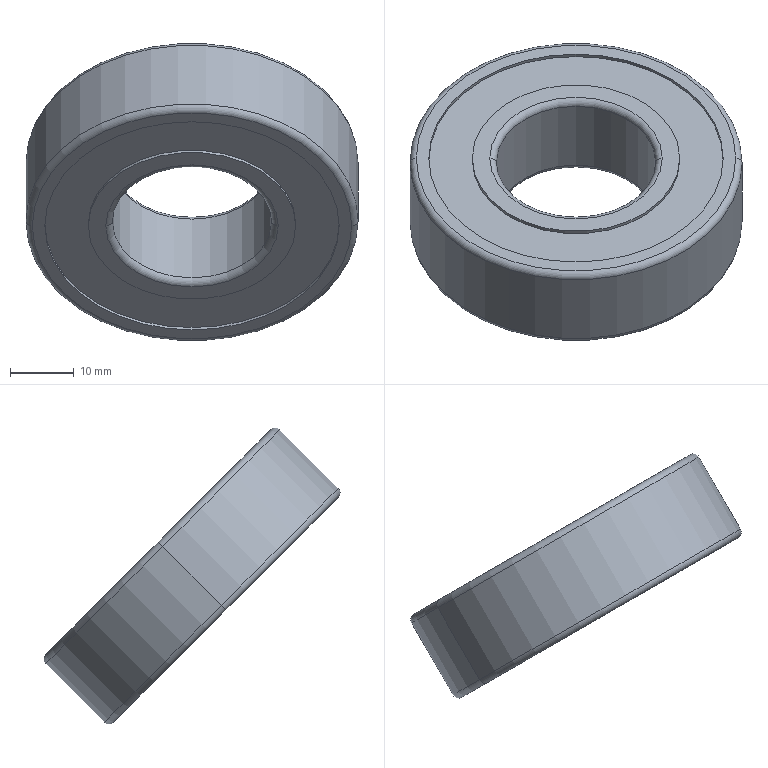Component | SolidWorks | PassiveRollerAssembly-1_Bearing6205-3 | 1 solid | 26 faces | box 52 x 46.55 x 46.55 mm | volume 23499 mm3 | cylinder 12 | torus 8 | plane 6 | commonest cylinder face diameters 46.1 x4 32.5 x4 52 x2 25 x2
build123d program:
from build123d import *


with BuildPart() as part:
    # Sketch1 → Revolve1 (revolve)
    with BuildSketch(Plane.XY, mode=Mode.PRIVATE) as revolve1_sk:
        with BuildLine():
            Line((0, 25), (0, 23.05))
            Line((0, 23.05), (0.53, 23.05))
            Line((0.53, 23.05), (0.53, 16.25))
            Line((0.53, 16.25), (0, 16.25))
            Line((0, 16.25), (0, 13.5))
            ThreePointArc((0, 13.5), (0.2929, 12.793), (1, 12.5))
            Line((1, 12.5), (14, 12.5))
            ThreePointArc((14, 12.5), (14.707, 12.793), (15, 13.5))
            Line((15, 13.5), (15, 16.25))
            Line((15, 16.25), (14.47, 16.25))
            Line((14.47, 16.25), (14.47, 23.05))
            Line((14.47, 23.05), (15, 23.05))
            Line((15, 23.05), (15, 25))
            ThreePointArc((15, 25), (14.707, 25.707), (14, 26))
            Line((14, 26), (1, 26))
            ThreePointArc((1, 26), (0.2929, 25.707), (0, 25))
        make_face()
    revolve(revolve1_sk.sketch.rotate(Axis((15, 0, 0), (-1, 0, 0)), 270), axis=Axis((15, 0, 0), (-1, 0, 0)))


solid = part.part

# Placed as in the assembly
solid = solid.moved(Location((2216.026, 747.574, 381.188), (-135, 89.432, 90)))
STEP:
#1=COLOUR_RGB('',0.7922,0.8196,0.9333);
#2=FILL_AREA_STYLE_COLOUR('',#1);
#3=FILL_AREA_STYLE('',(#2));
#4=SURFACE_STYLE_FILL_AREA(#3);
#5=SURFACE_SIDE_STYLE('',(#4));
#6=SURFACE_STYLE_USAGE(.BOTH.,#5);
#7=PRESENTATION_STYLE_ASSIGNMENT((#6));
#8=CARTESIAN_POINT('',(88.269,29.042,14.618));
#9=VERTEX_POINT('',#8);
#10=CARTESIAN_POINT('',(86.222,29.042,14.618));
#11=VERTEX_POINT('',#10);
#12=CARTESIAN_POINT('',(87.245,29.042,14.618));
#13=DIRECTION('',(-0.,0.7071,0.7071));
#14=DIRECTION('',(1.,0.,0.));
#15=AXIS2_PLACEMENT_3D('',#12,#13,#14);
#16=CIRCLE('',#15,1.024);
#17=EDGE_CURVE('',#9,#11,#16,.T.);
#18=ORIENTED_EDGE('',*,*,#17,.T.);
#19=CARTESIAN_POINT('',(86.222,29.404,14.98));
#20=VERTEX_POINT('',#19);
#21=CARTESIAN_POINT('',(86.222,29.014,14.59));
#22=DIRECTION('',(-0.,0.7071,0.7071));
#23=VECTOR('',#22,39.37);
#24=LINE('',#21,#23);
#25=EDGE_CURVE('',#11,#20,#24,.T.);
#26=ORIENTED_EDGE('',*,*,#25,.T.);
#27=CARTESIAN_POINT('',(88.269,29.404,14.98));
#28=VERTEX_POINT('',#27);
#29=CARTESIAN_POINT('',(87.245,29.404,14.98));
#30=DIRECTION('',(-0.,0.7071,0.7071));
#31=DIRECTION('',(1.,0.,0.));
#32=AXIS2_PLACEMENT_3D('',#29,#30,#31);
#33=CIRCLE('',#32,1.024);
#34=EDGE_CURVE('',#28,#20,#33,.T.);
#35=ORIENTED_EDGE('',*,*,#34,.F.);
#36=CARTESIAN_POINT('',(88.269,29.014,14.59));
#37=DIRECTION('',(-0.,0.7071,0.7071));
#38=VECTOR('',#37,39.37);
#39=LINE('',#36,#38);
#40=EDGE_CURVE('',#9,#28,#39,.T.);
#41=ORIENTED_EDGE('',*,*,#40,.F.);
#42=EDGE_LOOP('',(#18,#26,#35,#41));
#43=FACE_OUTER_BOUND('',#42,.T.);
#44=CARTESIAN_POINT('',(87.245,29.014,14.59));
#45=DIRECTION('',(-0.,0.7071,0.7071));
#46=DIRECTION('',(1.,0.,0.));
#47=AXIS2_PLACEMENT_3D('',#44,#45,#46);
#48=CYLINDRICAL_SURFACE('',#47,1.024);
#49=ADVANCED_FACE('',(#43),#48,.T.);
#50=CARTESIAN_POINT('',(88.229,29.014,14.59));
#51=VERTEX_POINT('',#50);
#52=CARTESIAN_POINT('',(86.261,29.014,14.59));
#53=VERTEX_POINT('',#52);
#54=CARTESIAN_POINT('',(87.245,29.014,14.59));
#55=DIRECTION('',(-0.,0.7071,0.7071));
#56=DIRECTION('',(1.,0.,0.));
#57=AXIS2_PLACEMENT_3D('',#54,#55,#56);
#58=CIRCLE('',#57,0.9843);
#59=EDGE_CURVE('',#51,#53,#58,.T.);
#60=ORIENTED_EDGE('',*,*,#59,.T.);
#61=CARTESIAN_POINT('',(86.261,29.042,14.618));
#62=DIRECTION('',(0.,0.7071,-0.7071));
#63=DIRECTION('',(0.,0.7071,0.7071));
#64=AXIS2_PLACEMENT_3D('',#61,#62,#63);
#65=CIRCLE('',#64,0.03937);
#66=EDGE_CURVE('',#53,#11,#65,.T.);
#67=ORIENTED_EDGE('',*,*,#66,.T.);
#68=ORIENTED_EDGE('',*,*,#17,.F.);
#69=CARTESIAN_POINT('',(88.229,29.042,14.618));
#70=DIRECTION('',(-0.,-0.7071,0.7071));
#71=DIRECTION('',(0.,-0.7071,-0.7071));
#72=AXIS2_PLACEMENT_3D('',#69,#70,#71);
#73=CIRCLE('',#72,0.03937);
#74=EDGE_CURVE('',#51,#9,#73,.T.);
#75=ORIENTED_EDGE('',*,*,#74,.F.);
#76=EDGE_LOOP('',(#60,#67,#68,#75));
#77=FACE_OUTER_BOUND('',#76,.T.);
#78=CARTESIAN_POINT('',(87.245,29.042,14.618));
#79=DIRECTION('',(-0.,0.7071,0.7071));
#80=DIRECTION('',(1.,0.,0.));
#81=AXIS2_PLACEMENT_3D('',#78,#79,#80);
#82=TOROIDAL_SURFACE('',#81,0.9843,0.03937);
#83=ADVANCED_FACE('',(#77),#82,.T.);
#84=CARTESIAN_POINT('',(86.338,29.014,14.59));
#85=VERTEX_POINT('',#84);
#86=CARTESIAN_POINT('',(88.153,29.014,14.59));
#87=VERTEX_POINT('',#86);
#88=CARTESIAN_POINT('',(87.245,29.014,14.59));
#89=DIRECTION('',(-0.,0.7071,0.7071));
#90=DIRECTION('',(1.,0.,0.));
#91=AXIS2_PLACEMENT_3D('',#88,#89,#90);
#92=CIRCLE('',#91,0.9075);
#93=EDGE_CURVE('',#85,#87,#92,.T.);
#94=ORIENTED_EDGE('',*,*,#93,.F.);
#95=CARTESIAN_POINT('',(86.338,29.029,14.605));
#96=VERTEX_POINT('',#95);
#97=CARTESIAN_POINT('',(86.338,29.014,14.59));
#98=DIRECTION('',(-0.,0.7071,0.7071));
#99=VECTOR('',#98,39.37);
#100=LINE('',#97,#99);
#101=EDGE_CURVE('',#85,#96,#100,.T.);
#102=ORIENTED_EDGE('',*,*,#101,.T.);
#103=CARTESIAN_POINT('',(88.153,29.029,14.605));
#104=VERTEX_POINT('',#103);
#105=CARTESIAN_POINT('',(87.245,29.029,14.605));
#106=DIRECTION('',(-0.,0.7071,0.7071));
#107=DIRECTION('',(1.,0.,0.));
#108=AXIS2_PLACEMENT_3D('',#105,#106,#107);
#109=CIRCLE('',#108,0.9075);
#110=EDGE_CURVE('',#96,#104,#109,.T.);
#111=ORIENTED_EDGE('',*,*,#110,.T.);
#112=CARTESIAN_POINT('',(88.153,29.014,14.59));
#113=DIRECTION('',(-0.,0.7071,0.7071));
#114=VECTOR('',#113,39.37);
#115=LINE('',#112,#114);
#116=EDGE_CURVE('',#87,#104,#115,.T.);
#117=ORIENTED_EDGE('',*,*,#116,.F.);
#118=EDGE_LOOP('',(#94,#102,#111,#117));
#119=FACE_OUTER_BOUND('',#118,.T.);
#120=CARTESIAN_POINT('',(87.245,29.014,14.59));
#121=DIRECTION('',(-0.,0.7071,0.7071));
#122=DIRECTION('',(1.,0.,0.));
#123=AXIS2_PLACEMENT_3D('',#120,#121,#122);
#124=CYLINDRICAL_SURFACE('',#123,0.9075);
#125=ADVANCED_FACE('',(#119),#124,.F.);
#126=CARTESIAN_POINT('',(87.885,29.014,14.59));
#127=VERTEX_POINT('',#126);
#128=CARTESIAN_POINT('',(86.605,29.014,14.59));
#129=VERTEX_POINT('',#128);
#130=CARTESIAN_POINT('',(87.245,29.014,14.59));
#131=DIRECTION('',(-0.,0.7071,0.7071));
#132=DIRECTION('',(1.,0.,0.));
#133=AXIS2_PLACEMENT_3D('',#130,#131,#132);
#134=CIRCLE('',#133,0.6398);
#135=EDGE_CURVE('',#127,#129,#134,.T.);
#136=ORIENTED_EDGE('',*,*,#135,.T.);
#137=CARTESIAN_POINT('',(86.605,29.029,14.605));
#138=VERTEX_POINT('',#137);
#139=CARTESIAN_POINT('',(86.605,29.014,14.59));
#140=DIRECTION('',(-0.,0.7071,0.7071));
#141=VECTOR('',#140,39.37);
#142=LINE('',#139,#141);
#143=EDGE_CURVE('',#129,#138,#142,.T.);
#144=ORIENTED_EDGE('',*,*,#143,.T.);
#145=CARTESIAN_POINT('',(87.885,29.029,14.605));
#146=VERTEX_POINT('',#145);
#147=CARTESIAN_POINT('',(87.245,29.029,14.605));
#148=DIRECTION('',(-0.,0.7071,0.7071));
#149=DIRECTION('',(1.,0.,0.));
#150=AXIS2_PLACEMENT_3D('',#147,#148,#149);
#151=CIRCLE('',#150,0.6398);
#152=EDGE_CURVE('',#146,#138,#151,.T.);
#153=ORIENTED_EDGE('',*,*,#152,.F.);
#154=CARTESIAN_POINT('',(87.885,29.014,14.59));
#155=DIRECTION('',(-0.,0.7071,0.7071));
#156=VECTOR('',#155,39.37);
#157=LINE('',#154,#156);
#158=EDGE_CURVE('',#127,#146,#157,.T.);
#159=ORIENTED_EDGE('',*,*,#158,.F.);
#160=EDGE_LOOP('',(#136,#144,#153,#159));
#161=FACE_OUTER_BOUND('',#160,.T.);
#162=CARTESIAN_POINT('',(87.245,29.014,14.59));
#163=DIRECTION('',(-0.,0.7071,0.7071));
#164=DIRECTION('',(1.,0.,0.));
#165=AXIS2_PLACEMENT_3D('',#162,#163,#164);
#166=CYLINDRICAL_SURFACE('',#165,0.6398);
#167=ADVANCED_FACE('',(#161),#166,.T.);
#168=CARTESIAN_POINT('',(87.737,29.042,14.618));
#169=VERTEX_POINT('',#168);
#170=CARTESIAN_POINT('',(86.753,29.042,14.618));
#171=VERTEX_POINT('',#170);
#172=CARTESIAN_POINT('',(87.245,29.042,14.618));
#173=DIRECTION('',(-0.,0.7071,0.7071));
#174=DIRECTION('',(1.,0.,0.));
#175=AXIS2_PLACEMENT_3D('',#172,#173,#174);
#176=CIRCLE('',#175,0.4921);
#177=EDGE_CURVE('',#169,#171,#176,.T.);
#178=ORIENTED_EDGE('',*,*,#177,.T.);
#179=CARTESIAN_POINT('',(86.714,29.014,14.59));
#180=VERTEX_POINT('',#179);
#181=CARTESIAN_POINT('',(86.714,29.042,14.618));
#182=DIRECTION('',(0.,0.7071,-0.7071));
#183=DIRECTION('',(0.,0.7071,0.7071));
#184=AXIS2_PLACEMENT_3D('',#181,#182,#183);
#185=CIRCLE('',#184,0.03937);
#186=EDGE_CURVE('',#171,#180,#185,.T.);
#187=ORIENTED_EDGE('',*,*,#186,.T.);
#188=CARTESIAN_POINT('',(87.777,29.014,14.59));
#189=VERTEX_POINT('',#188);
#190=CARTESIAN_POINT('',(87.245,29.014,14.59));
#191=DIRECTION('',(-0.,0.7071,0.7071));
#192=DIRECTION('',(1.,0.,0.));
#193=AXIS2_PLACEMENT_3D('',#190,#191,#192);
#194=CIRCLE('',#193,0.5315);
#195=EDGE_CURVE('',#189,#180,#194,.T.);
#196=ORIENTED_EDGE('',*,*,#195,.F.);
#197=CARTESIAN_POINT('',(87.777,29.042,14.618));
#198=DIRECTION('',(-0.,-0.7071,0.7071));
#199=DIRECTION('',(0.,-0.7071,-0.7071));
#200=AXIS2_PLACEMENT_3D('',#197,#198,#199);
#201=CIRCLE('',#200,0.03937);
#202=EDGE_CURVE('',#169,#189,#201,.T.);
#203=ORIENTED_EDGE('',*,*,#202,.F.);
#204=EDGE_LOOP('',(#178,#187,#196,#203));
#205=FACE_OUTER_BOUND('',#204,.T.);
#206=CARTESIAN_POINT('',(87.245,29.042,14.618));
#207=DIRECTION('',(-0.,0.7071,0.7071));
#208=DIRECTION('',(1.,0.,0.));
#209=AXIS2_PLACEMENT_3D('',#206,#207,#208);
#210=TOROIDAL_SURFACE('',#209,0.5315,0.03937);
#211=ADVANCED_FACE('',(#205),#210,.T.);
#212=CARTESIAN_POINT('',(87.245,29.042,14.618));
#213=DIRECTION('',(-0.,0.7071,0.7071));
#214=DIRECTION('',(1.,0.,0.));
#215=AXIS2_PLACEMENT_3D('',#212,#213,#214);
#216=CIRCLE('',#215,0.4921);
#217=EDGE_CURVE('',#171,#169,#216,.T.);
#218=ORIENTED_EDGE('',*,*,#217,.F.);
#219=CARTESIAN_POINT('',(86.753,29.404,14.98));
#220=VERTEX_POINT('',#219);
#221=CARTESIAN_POINT('',(86.753,29.014,14.59));
#222=DIRECTION('',(-0.,0.7071,0.7071));
#223=VECTOR('',#222,39.37);
#224=LINE('',#221,#223);
#225=EDGE_CURVE('',#171,#220,#224,.T.);
#226=ORIENTED_EDGE('',*,*,#225,.T.);
#227=CARTESIAN_POINT('',(87.737,29.404,14.98));
#228=VERTEX_POINT('',#227);
#229=CARTESIAN_POINT('',(87.245,29.404,14.98));
#230=DIRECTION('',(-0.,0.7071,0.7071));
#231=DIRECTION('',(1.,0.,0.));
#232=AXIS2_PLACEMENT_3D('',#229,#230,#231);
#233=CIRCLE('',#232,0.4921);
#234=EDGE_CURVE('',#220,#228,#233,.T.);
#235=ORIENTED_EDGE('',*,*,#234,.T.);
#236=CARTESIAN_POINT('',(87.737,29.014,14.59));
#237=DIRECTION('',(-0.,0.7071,0.7071));
#238=VECTOR('',#237,39.37);
#239=LINE('',#236,#238);
#240=EDGE_CURVE('',#169,#228,#239,.T.);
#241=ORIENTED_EDGE('',*,*,#240,.F.);
#242=EDGE_LOOP('',(#218,#226,#235,#241));
#243=FACE_OUTER_BOUND('',#242,.T.);
#244=CARTESIAN_POINT('',(87.245,29.014,14.59));
#245=DIRECTION('',(-0.,0.7071,0.7071));
#246=DIRECTION('',(1.,0.,0.));
#247=AXIS2_PLACEMENT_3D('',#244,#245,#246);
#248=CYLINDRICAL_SURFACE('',#247,0.4921);
#249=ADVANCED_FACE('',(#243),#248,.F.);
#250=CARTESIAN_POINT('',(87.777,29.432,15.007));
#251=VERTEX_POINT('',#250);
#252=CARTESIAN_POINT('',(86.714,29.432,15.007));
#253=VERTEX_POINT('',#252);
#254=CARTESIAN_POINT('',(87.245,29.432,15.007));
#255=DIRECTION('',(-0.,0.7071,0.7071));
#256=DIRECTION('',(1.,0.,0.));
#257=AXIS2_PLACEMENT_3D('',#254,#255,#256);
#258=CIRCLE('',#257,0.5315);
#259=EDGE_CURVE('',#251,#253,#258,.T.);
#260=ORIENTED_EDGE('',*,*,#259,.T.);
#261=CARTESIAN_POINT('',(86.714,29.404,14.98));
#262=DIRECTION('',(0.,0.7071,-0.7071));
#263=DIRECTION('',(0.,0.7071,0.7071));
#264=AXIS2_PLACEMENT_3D('',#261,#262,#263);
#265=CIRCLE('',#264,0.03937);
#266=EDGE_CURVE('',#253,#220,#265,.T.);
#267=ORIENTED_EDGE('',*,*,#266,.T.);
#268=CARTESIAN_POINT('',(87.245,29.404,14.98));
#269=DIRECTION('',(-0.,0.7071,0.7071));
#270=DIRECTION('',(1.,0.,0.));
#271=AXIS2_PLACEMENT_3D('',#268,#269,#270);
#272=CIRCLE('',#271,0.4921);
#273=EDGE_CURVE('',#228,#220,#272,.T.);
#274=ORIENTED_EDGE('',*,*,#273,.F.);
#275=CARTESIAN_POINT('',(87.777,29.404,14.98));
#276=DIRECTION('',(-0.,-0.7071,0.7071));
#277=DIRECTION('',(0.,-0.7071,-0.7071));
#278=AXIS2_PLACEMENT_3D('',#275,#276,#277);
#279=CIRCLE('',#278,0.03937);
#280=EDGE_CURVE('',#251,#228,#279,.T.);
#281=ORIENTED_EDGE('',*,*,#280,.F.);
#282=EDGE_LOOP('',(#260,#267,#274,#281));
#283=FACE_OUTER_BOUND('',#282,.T.);
#284=CARTESIAN_POINT('',(87.245,29.404,14.98));
#285=DIRECTION('',(-0.,0.7071,0.7071));
#286=DIRECTION('',(1.,0.,0.));
#287=AXIS2_PLACEMENT_3D('',#284,#285,#286);
#288=TOROIDAL_SURFACE('',#287,0.5315,0.03937);
#289=ADVANCED_FACE('',(#283),#288,.T.);
#290=CARTESIAN_POINT('',(87.885,29.417,14.993));
#291=VERTEX_POINT('',#290);
#292=CARTESIAN_POINT('',(86.605,29.417,14.993));
#293=VERTEX_POINT('',#292);
#294=CARTESIAN_POINT('',(87.245,29.417,14.993));
#295=DIRECTION('',(-0.,0.7071,0.7071));
#296=DIRECTION('',(1.,0.,0.));
#297=AXIS2_PLACEMENT_3D('',#294,#295,#296);
#298=CIRCLE('',#297,0.6398);
#299=EDGE_CURVE('',#291,#293,#298,.T.);
#300=ORIENTED_EDGE('',*,*,#299,.T.);
#301=CARTESIAN_POINT('',(86.605,29.432,15.007));
#302=VERTEX_POINT('',#301);
#303=CARTESIAN_POINT('',(86.605,29.014,14.59));
#304=DIRECTION('',(-0.,0.7071,0.7071));
#305=VECTOR('',#304,39.37);
#306=LINE('',#303,#305);
#307=EDGE_CURVE('',#293,#302,#306,.T.);
#308=ORIENTED_EDGE('',*,*,#307,.T.);
#309=CARTESIAN_POINT('',(87.885,29.432,15.007));
#310=VERTEX_POINT('',#309);
#311=CARTESIAN_POINT('',(87.245,29.432,15.007));
#312=DIRECTION('',(-0.,0.7071,0.7071));
#313=DIRECTION('',(1.,0.,0.));
#314=AXIS2_PLACEMENT_3D('',#311,#312,#313);
#315=CIRCLE('',#314,0.6398);
#316=EDGE_CURVE('',#310,#302,#315,.T.);
#317=ORIENTED_EDGE('',*,*,#316,.F.);
#318=CARTESIAN_POINT('',(87.885,29.014,14.59));
#319=DIRECTION('',(-0.,0.7071,0.7071));
#320=VECTOR('',#319,39.37);
#321=LINE('',#318,#320);
#322=EDGE_CURVE('',#291,#310,#321,.T.);
#323=ORIENTED_EDGE('',*,*,#322,.F.);
#324=EDGE_LOOP('',(#300,#308,#317,#323));
#325=FACE_OUTER_BOUND('',#324,.T.);
#326=CARTESIAN_POINT('',(87.245,29.014,14.59));
#327=DIRECTION('',(-0.,0.7071,0.7071));
#328=DIRECTION('',(1.,0.,0.));
#329=AXIS2_PLACEMENT_3D('',#326,#327,#328);
#330=CYLINDRICAL_SURFACE('',#329,0.6398);
#331=ADVANCED_FACE('',(#325),#330,.T.);
#332=CARTESIAN_POINT('',(86.338,29.417,14.993));
#333=VERTEX_POINT('',#332);
#334=CARTESIAN_POINT('',(88.153,29.417,14.993));
#335=VERTEX_POINT('',#334);
#336=CARTESIAN_POINT('',(87.245,29.417,14.993));
#337=DIRECTION('',(-0.,0.7071,0.7071));
#338=DIRECTION('',(1.,0.,0.));
#339=AXIS2_PLACEMENT_3D('',#336,#337,#338);
#340=CIRCLE('',#339,0.9075);
#341=EDGE_CURVE('',#333,#335,#340,.T.);
#342=ORIENTED_EDGE('',*,*,#341,.F.);
#343=CARTESIAN_POINT('',(86.338,29.432,15.007));
#344=VERTEX_POINT('',#343);
#345=CARTESIAN_POINT('',(86.338,29.014,14.59));
#346=DIRECTION('',(-0.,0.7071,0.7071));
#347=VECTOR('',#346,39.37);
#348=LINE('',#345,#347);
#349=EDGE_CURVE('',#333,#344,#348,.T.);
#350=ORIENTED_EDGE('',*,*,#349,.T.);
#351=CARTESIAN_POINT('',(88.153,29.432,15.007));
#352=VERTEX_POINT('',#351);
#353=CARTESIAN_POINT('',(87.245,29.432,15.007));
#354=DIRECTION('',(-0.,0.7071,0.7071));
#355=DIRECTION('',(1.,0.,0.));
#356=AXIS2_PLACEMENT_3D('',#353,#354,#355);
#357=CIRCLE('',#356,0.9075);
#358=EDGE_CURVE('',#344,#352,#357,.T.);
#359=ORIENTED_EDGE('',*,*,#358,.T.);
#360=CARTESIAN_POINT('',(88.153,29.014,14.59));
#361=DIRECTION('',(-0.,0.7071,0.7071));
#362=VECTOR('',#361,39.37);
#363=LINE('',#360,#362);
#364=EDGE_CURVE('',#335,#352,#363,.T.);
#365=ORIENTED_EDGE('',*,*,#364,.F.);
#366=EDGE_LOOP('',(#342,#350,#359,#365));
#367=FACE_OUTER_BOUND('',#366,.T.);
#368=CARTESIAN_POINT('',(87.245,29.014,14.59));
#369=DIRECTION('',(-0.,0.7071,0.7071));
#370=DIRECTION('',(1.,0.,0.));
#371=AXIS2_PLACEMENT_3D('',#368,#369,#370);
#372=CYLINDRICAL_SURFACE('',#371,0.9075);
#373=ADVANCED_FACE('',(#367),#372,.F.);
#374=ORIENTED_EDGE('',*,*,#34,.T.);
#375=CARTESIAN_POINT('',(86.261,29.432,15.007));
#376=VERTEX_POINT('',#375);
#377=CARTESIAN_POINT('',(86.261,29.404,14.98));
#378=DIRECTION('',(0.,0.7071,-0.7071));
#379=DIRECTION('',(0.,0.7071,0.7071));
#380=AXIS2_PLACEMENT_3D('',#377,#378,#379);
#381=CIRCLE('',#380,0.03937);
#382=EDGE_CURVE('',#20,#376,#381,.T.);
#383=ORIENTED_EDGE('',*,*,#382,.T.);
#384=CARTESIAN_POINT('',(88.229,29.432,15.007));
#385=VERTEX_POINT('',#384);
#386=CARTESIAN_POINT('',(87.245,29.432,15.007));
#387=DIRECTION('',(-0.,0.7071,0.7071));
#388=DIRECTION('',(1.,0.,0.));
#389=AXIS2_PLACEMENT_3D('',#386,#387,#388);
#390=CIRCLE('',#389,0.9843);
#391=EDGE_CURVE('',#385,#376,#390,.T.);
#392=ORIENTED_EDGE('',*,*,#391,.F.);
#393=CARTESIAN_POINT('',(88.229,29.404,14.98));
#394=DIRECTION('',(-0.,-0.7071,0.7071));
#395=DIRECTION('',(0.,-0.7071,-0.7071));
#396=AXIS2_PLACEMENT_3D('',#393,#394,#395);
#397=CIRCLE('',#396,0.03937);
#398=EDGE_CURVE('',#28,#385,#397,.T.);
#399=ORIENTED_EDGE('',*,*,#398,.F.);
#400=EDGE_LOOP('',(#374,#383,#392,#399));
#401=FACE_OUTER_BOUND('',#400,.T.);
#402=CARTESIAN_POINT('',(87.245,29.404,14.98));
#403=DIRECTION('',(-0.,0.7071,0.7071));
#404=DIRECTION('',(1.,0.,0.));
#405=AXIS2_PLACEMENT_3D('',#402,#403,#404);
#406=TOROIDAL_SURFACE('',#405,0.9843,0.03937);
#407=ADVANCED_FACE('',(#401),#406,.T.);
#408=ORIENTED_EDGE('',*,*,#382,.F.);
#409=CARTESIAN_POINT('',(87.245,29.404,14.98));
#410=DIRECTION('',(-0.,0.7071,0.7071));
#411=DIRECTION('',(1.,0.,0.));
#412=AXIS2_PLACEMENT_3D('',#409,#410,#411);
#413=CIRCLE('',#412,1.024);
#414=EDGE_CURVE('',#20,#28,#413,.T.);
#415=ORIENTED_EDGE('',*,*,#414,.T.);
#416=ORIENTED_EDGE('',*,*,#398,.T.);
#417=CARTESIAN_POINT('',(87.245,29.432,15.007));
#418=DIRECTION('',(-0.,0.7071,0.7071));
#419=DIRECTION('',(1.,0.,0.));
#420=AXIS2_PLACEMENT_3D('',#417,#418,#419);
#421=CIRCLE('',#420,0.9843);
#422=EDGE_CURVE('',#376,#385,#421,.T.);
#423=ORIENTED_EDGE('',*,*,#422,.F.);
#424=EDGE_LOOP('',(#408,#415,#416,#423));
#425=FACE_OUTER_BOUND('',#424,.T.);
#426=CARTESIAN_POINT('',(87.245,29.404,14.98));
#427=DIRECTION('',(-0.,0.7071,0.7071));
#428=DIRECTION('',(1.,0.,0.));
#429=AXIS2_PLACEMENT_3D('',#426,#427,#428);
#430=TOROIDAL_SURFACE('',#429,0.9843,0.03937);
#431=ADVANCED_FACE('',(#425),#430,.T.);
#432=CARTESIAN_POINT('',(87.245,29.432,15.007));
#433=DIRECTION('',(-0.,0.7071,0.7071));
#434=DIRECTION('',(1.,0.,0.));
#435=AXIS2_PLACEMENT_3D('',#432,#433,#434);
#436=CIRCLE('',#435,0.9075);
#437=EDGE_CURVE('',#352,#344,#436,.T.);
#438=ORIENTED_EDGE('',*,*,#437,.F.);
#439=ORIENTED_EDGE('',*,*,#358,.F.);
#440=EDGE_LOOP('',(#438,#439));
#441=FACE_BOUND('',#440,.T.);
#442=ORIENTED_EDGE('',*,*,#391,.T.);
#443=ORIENTED_EDGE('',*,*,#422,.T.);
#444=EDGE_LOOP('',(#442,#443));
#445=FACE_OUTER_BOUND('',#444,.T.);
#446=CARTESIAN_POINT('',(87.245,30.128,14.311));
#447=DIRECTION('',(0.,-0.7071,-0.7071));
#448=DIRECTION('',(-1.,-0.,-0.));
#449=AXIS2_PLACEMENT_3D('',#446,#447,#448);
#450=PLANE('',#449);
#451=ADVANCED_FACE('',(#441,#445),#450,.F.);
#452=ORIENTED_EDGE('',*,*,#349,.F.);
#453=CARTESIAN_POINT('',(87.245,29.417,14.993));
#454=DIRECTION('',(-0.,0.7071,0.7071));
#455=DIRECTION('',(1.,0.,0.));
#456=AXIS2_PLACEMENT_3D('',#453,#454,#455);
#457=CIRCLE('',#456,0.9075);
#458=EDGE_CURVE('',#335,#333,#457,.T.);
#459=ORIENTED_EDGE('',*,*,#458,.F.);
#460=ORIENTED_EDGE('',*,*,#364,.T.);
#461=ORIENTED_EDGE('',*,*,#437,.T.);
#462=EDGE_LOOP('',(#452,#459,#460,#461));
#463=FACE_OUTER_BOUND('',#462,.T.);
#464=CARTESIAN_POINT('',(87.245,29.014,14.59));
#465=DIRECTION('',(-0.,0.7071,0.7071));
#466=DIRECTION('',(1.,0.,0.));
#467=AXIS2_PLACEMENT_3D('',#464,#465,#466);
#468=CYLINDRICAL_SURFACE('',#467,0.9075);
#469=ADVANCED_FACE('',(#463),#468,.F.);
#470=ORIENTED_EDGE('',*,*,#299,.F.);
#471=CARTESIAN_POINT('',(87.245,29.417,14.993));
#472=DIRECTION('',(-0.,0.7071,0.7071));
#473=DIRECTION('',(1.,0.,0.));
#474=AXIS2_PLACEMENT_3D('',#471,#472,#473);
#475=CIRCLE('',#474,0.6398);
#476=EDGE_CURVE('',#293,#291,#475,.T.);
#477=ORIENTED_EDGE('',*,*,#476,.F.);
#478=EDGE_LOOP('',(#470,#477));
#479=FACE_BOUND('',#478,.T.);
#480=ORIENTED_EDGE('',*,*,#458,.T.);
#481=ORIENTED_EDGE('',*,*,#341,.T.);
#482=EDGE_LOOP('',(#480,#481));
#483=FACE_OUTER_BOUND('',#482,.T.);
#484=CARTESIAN_POINT('',(87.245,30.059,14.351));
#485=DIRECTION('',(0.,-0.7071,-0.7071));
#486=DIRECTION('',(-1.,-0.,-0.));
#487=AXIS2_PLACEMENT_3D('',#484,#485,#486);
#488=PLANE('',#487);
#489=ADVANCED_FACE('',(#479,#483),#488,.F.);
#490=ORIENTED_EDGE('',*,*,#307,.F.);
#491=ORIENTED_EDGE('',*,*,#476,.T.);
#492=ORIENTED_EDGE('',*,*,#322,.T.);
#493=CARTESIAN_POINT('',(87.245,29.432,15.007));
#494=DIRECTION('',(-0.,0.7071,0.7071));
#495=DIRECTION('',(1.,0.,0.));
#496=AXIS2_PLACEMENT_3D('',#493,#494,#495);
#497=CIRCLE('',#496,0.6398);
#498=EDGE_CURVE('',#302,#310,#497,.T.);
#499=ORIENTED_EDGE('',*,*,#498,.F.);
#500=EDGE_LOOP('',(#490,#491,#492,#499));
#501=FACE_OUTER_BOUND('',#500,.T.);
#502=CARTESIAN_POINT('',(87.245,29.014,14.59));
#503=DIRECTION('',(-0.,0.7071,0.7071));
#504=DIRECTION('',(1.,0.,0.));
#505=AXIS2_PLACEMENT_3D('',#502,#503,#504);
#506=CYLINDRICAL_SURFACE('',#505,0.6398);
#507=ADVANCED_FACE('',(#501),#506,.T.);
#508=ORIENTED_EDGE('',*,*,#259,.F.);
#509=CARTESIAN_POINT('',(87.245,29.432,15.007));
#510=DIRECTION('',(-0.,0.7071,0.7071));
#511=DIRECTION('',(1.,0.,0.));
#512=AXIS2_PLACEMENT_3D('',#509,#510,#511);
#513=CIRCLE('',#512,0.5315);
#514=EDGE_CURVE('',#253,#251,#513,.T.);
#515=ORIENTED_EDGE('',*,*,#514,.F.);
#516=EDGE_LOOP('',(#508,#515));
#517=FACE_BOUND('',#516,.T.);
#518=ORIENTED_EDGE('',*,*,#316,.T.);
#519=ORIENTED_EDGE('',*,*,#498,.T.);
#520=EDGE_LOOP('',(#518,#519));
#521=FACE_OUTER_BOUND('',#520,.T.);
#522=CARTESIAN_POINT('',(87.245,29.884,14.555));
#523=DIRECTION('',(0.,-0.7071,-0.7071));
#524=DIRECTION('',(-1.,-0.,-0.));
#525=AXIS2_PLACEMENT_3D('',#522,#523,#524);
#526=PLANE('',#525);
#527=ADVANCED_FACE('',(#517,#521),#526,.F.);
#528=ORIENTED_EDGE('',*,*,#266,.F.);
#529=ORIENTED_EDGE('',*,*,#514,.T.);
#530=ORIENTED_EDGE('',*,*,#280,.T.);
#531=ORIENTED_EDGE('',*,*,#234,.F.);
#532=EDGE_LOOP('',(#528,#529,#530,#531));
#533=FACE_OUTER_BOUND('',#532,.T.);
#534=CARTESIAN_POINT('',(87.245,29.404,14.98));
#535=DIRECTION('',(-0.,0.7071,0.7071));
#536=DIRECTION('',(1.,0.,0.));
#537=AXIS2_PLACEMENT_3D('',#534,#535,#536);
#538=TOROIDAL_SURFACE('',#537,0.5315,0.03937);
#539=ADVANCED_FACE('',(#533),#538,.T.);
#540=ORIENTED_EDGE('',*,*,#225,.F.);
#541=ORIENTED_EDGE('',*,*,#177,.F.);
#542=ORIENTED_EDGE('',*,*,#240,.T.);
#543=ORIENTED_EDGE('',*,*,#273,.T.);
#544=EDGE_LOOP('',(#540,#541,#542,#543));
#545=FACE_OUTER_BOUND('',#544,.T.);
#546=CARTESIAN_POINT('',(87.245,29.014,14.59));
#547=DIRECTION('',(-0.,0.7071,0.7071));
#548=DIRECTION('',(1.,0.,0.));
#549=AXIS2_PLACEMENT_3D('',#546,#547,#548);
#550=CYLINDRICAL_SURFACE('',#549,0.4921);
#551=ADVANCED_FACE('',(#545),#550,.F.);
#552=ORIENTED_EDGE('',*,*,#186,.F.);
#553=ORIENTED_EDGE('',*,*,#217,.T.);
#554=ORIENTED_EDGE('',*,*,#202,.T.);
#555=CARTESIAN_POINT('',(87.245,29.014,14.59));
#556=DIRECTION('',(-0.,0.7071,0.7071));
#557=DIRECTION('',(1.,0.,0.));
#558=AXIS2_PLACEMENT_3D('',#555,#556,#557);
#559=CIRCLE('',#558,0.5315);
#560=EDGE_CURVE('',#180,#189,#559,.T.);
#561=ORIENTED_EDGE('',*,*,#560,.F.);
#562=EDGE_LOOP('',(#552,#553,#554,#561));
#563=FACE_OUTER_BOUND('',#562,.T.);
#564=CARTESIAN_POINT('',(87.245,29.042,14.618));
#565=DIRECTION('',(-0.,0.7071,0.7071));
#566=DIRECTION('',(1.,0.,0.));
#567=AXIS2_PLACEMENT_3D('',#564,#565,#566);
#568=TOROIDAL_SURFACE('',#567,0.5315,0.03937);
#569=ADVANCED_FACE('',(#563),#568,.T.);
#570=ORIENTED_EDGE('',*,*,#135,.F.);
#571=CARTESIAN_POINT('',(87.245,29.014,14.59));
#572=DIRECTION('',(-0.,0.7071,0.7071));
#573=DIRECTION('',(1.,0.,0.));
#574=AXIS2_PLACEMENT_3D('',#571,#572,#573);
#575=CIRCLE('',#574,0.6398);
#576=EDGE_CURVE('',#129,#127,#575,.T.);
#577=ORIENTED_EDGE('',*,*,#576,.F.);
#578=EDGE_LOOP('',(#570,#577));
#579=FACE_OUTER_BOUND('',#578,.T.);
#580=ORIENTED_EDGE('',*,*,#195,.T.);
#581=ORIENTED_EDGE('',*,*,#560,.T.);
#582=EDGE_LOOP('',(#580,#581));
#583=FACE_BOUND('',#582,.T.);
#584=CARTESIAN_POINT('',(87.245,29.39,14.214));
#585=DIRECTION('',(-0.,0.7071,0.7071));
#586=DIRECTION('',(1.,0.,0.));
#587=AXIS2_PLACEMENT_3D('',#584,#585,#586);
#588=PLANE('',#587);
#589=ADVANCED_FACE('',(#579,#583),#588,.F.);
#590=ORIENTED_EDGE('',*,*,#143,.F.);
#591=ORIENTED_EDGE('',*,*,#576,.T.);
#592=ORIENTED_EDGE('',*,*,#158,.T.);
#593=CARTESIAN_POINT('',(87.245,29.029,14.605));
#594=DIRECTION('',(-0.,0.7071,0.7071));
#595=DIRECTION('',(1.,0.,0.));
#596=AXIS2_PLACEMENT_3D('',#593,#594,#595);
#597=CIRCLE('',#596,0.6398);
#598=EDGE_CURVE('',#138,#146,#597,.T.);
#599=ORIENTED_EDGE('',*,*,#598,.F.);
#600=EDGE_LOOP('',(#590,#591,#592,#599));
#601=FACE_OUTER_BOUND('',#600,.T.);
#602=CARTESIAN_POINT('',(87.245,29.014,14.59));
#603=DIRECTION('',(-0.,0.7071,0.7071));
#604=DIRECTION('',(1.,0.,0.));
#605=AXIS2_PLACEMENT_3D('',#602,#603,#604);
#606=CYLINDRICAL_SURFACE('',#605,0.6398);
#607=ADVANCED_FACE('',(#601),#606,.T.);
#608=CARTESIAN_POINT('',(87.245,29.029,14.605));
#609=DIRECTION('',(-0.,0.7071,0.7071));
#610=DIRECTION('',(1.,0.,0.));
#611=AXIS2_PLACEMENT_3D('',#608,#609,#610);
#612=CIRCLE('',#611,0.9075);
#613=EDGE_CURVE('',#104,#96,#612,.T.);
#614=ORIENTED_EDGE('',*,*,#613,.F.);
#615=ORIENTED_EDGE('',*,*,#110,.F.);
#616=EDGE_LOOP('',(#614,#615));
#617=FACE_OUTER_BOUND('',#616,.T.);
#618=ORIENTED_EDGE('',*,*,#152,.T.);
#619=ORIENTED_EDGE('',*,*,#598,.T.);
#620=EDGE_LOOP('',(#618,#619));
#621=FACE_BOUND('',#620,.T.);
#622=CARTESIAN_POINT('',(87.245,29.482,14.152));
#623=DIRECTION('',(-0.,0.7071,0.7071));
#624=DIRECTION('',(1.,0.,0.));
#625=AXIS2_PLACEMENT_3D('',#622,#623,#624);
#626=PLANE('',#625);
#627=ADVANCED_FACE('',(#617,#621),#626,.F.);
#628=ORIENTED_EDGE('',*,*,#101,.F.);
#629=CARTESIAN_POINT('',(87.245,29.014,14.59));
#630=DIRECTION('',(-0.,0.7071,0.7071));
#631=DIRECTION('',(1.,0.,0.));
#632=AXIS2_PLACEMENT_3D('',#629,#630,#631);
#633=CIRCLE('',#632,0.9075);
#634=EDGE_CURVE('',#87,#85,#633,.T.);
#635=ORIENTED_EDGE('',*,*,#634,.F.);
#636=ORIENTED_EDGE('',*,*,#116,.T.);
#637=ORIENTED_EDGE('',*,*,#613,.T.);
#638=EDGE_LOOP('',(#628,#635,#636,#637));
#639=FACE_OUTER_BOUND('',#638,.T.);
#640=CARTESIAN_POINT('',(87.245,29.014,14.59));
#641=DIRECTION('',(-0.,0.7071,0.7071));
#642=DIRECTION('',(1.,0.,0.));
#643=AXIS2_PLACEMENT_3D('',#640,#641,#642);
#644=CYLINDRICAL_SURFACE('',#643,0.9075);
#645=ADVANCED_FACE('',(#639),#644,.F.);
#646=ORIENTED_EDGE('',*,*,#59,.F.);
#647=CARTESIAN_POINT('',(87.245,29.014,14.59));
#648=DIRECTION('',(-0.,0.7071,0.7071));
#649=DIRECTION('',(1.,0.,0.));
#650=AXIS2_PLACEMENT_3D('',#647,#648,#649);
#651=CIRCLE('',#650,0.9843);
#652=EDGE_CURVE('',#53,#51,#651,.T.);
#653=ORIENTED_EDGE('',*,*,#652,.F.);
#654=EDGE_LOOP('',(#646,#653));
#655=FACE_OUTER_BOUND('',#654,.T.);
#656=ORIENTED_EDGE('',*,*,#634,.T.);
#657=ORIENTED_EDGE('',*,*,#93,.T.);
#658=EDGE_LOOP('',(#656,#657));
#659=FACE_BOUND('',#658,.T.);
#660=CARTESIAN_POINT('',(87.245,29.656,13.948));
#661=DIRECTION('',(-0.,0.7071,0.7071));
#662=DIRECTION('',(1.,0.,0.));
#663=AXIS2_PLACEMENT_3D('',#660,#661,#662);
#664=PLANE('',#663);
#665=ADVANCED_FACE('',(#655,#659),#664,.F.);
#666=ORIENTED_EDGE('',*,*,#66,.F.);
#667=ORIENTED_EDGE('',*,*,#652,.T.);
#668=ORIENTED_EDGE('',*,*,#74,.T.);
#669=CARTESIAN_POINT('',(87.245,29.042,14.618));
#670=DIRECTION('',(-0.,0.7071,0.7071));
#671=DIRECTION('',(1.,0.,0.));
#672=AXIS2_PLACEMENT_3D('',#669,#670,#671);
#673=CIRCLE('',#672,1.024);
#674=EDGE_CURVE('',#11,#9,#673,.T.);
#675=ORIENTED_EDGE('',*,*,#674,.F.);
#676=EDGE_LOOP('',(#666,#667,#668,#675));
#677=FACE_OUTER_BOUND('',#676,.T.);
#678=CARTESIAN_POINT('',(87.245,29.042,14.618));
#679=DIRECTION('',(-0.,0.7071,0.7071));
#680=DIRECTION('',(1.,0.,0.));
#681=AXIS2_PLACEMENT_3D('',#678,#679,#680);
#682=TOROIDAL_SURFACE('',#681,0.9843,0.03937);
#683=ADVANCED_FACE('',(#677),#682,.T.);
#684=ORIENTED_EDGE('',*,*,#25,.F.);
#685=ORIENTED_EDGE('',*,*,#674,.T.);
#686=ORIENTED_EDGE('',*,*,#40,.T.);
#687=ORIENTED_EDGE('',*,*,#414,.F.);
#688=EDGE_LOOP('',(#684,#685,#686,#687));
#689=FACE_OUTER_BOUND('',#688,.T.);
#690=CARTESIAN_POINT('',(87.245,29.014,14.59));
#691=DIRECTION('',(-0.,0.7071,0.7071));
#692=DIRECTION('',(1.,0.,0.));
#693=AXIS2_PLACEMENT_3D('',#690,#691,#692);
#694=CYLINDRICAL_SURFACE('',#693,1.024);
#695=ADVANCED_FACE('',(#689),#694,.T.);
#696=CLOSED_SHELL('',(#49,#83,#125,#167,#211,#249,#289,#331,#373,#407,#431,#451,#469,#489,#507,#527,#539,#551,#569,#589,#607,#627,#645,#665,#683,#695));
#697=MANIFOLD_SOLID_BREP('',#696);
#698=STYLED_ITEM('',(#7),#697);
#699=(LENGTH_UNIT()NAMED_UNIT(*)SI_UNIT($,.METRE.));
#700=LENGTH_MEASURE_WITH_UNIT(LENGTH_MEASURE(0.0254),#699);
#701=DIMENSIONAL_EXPONENTS(1.,0.,0.,0.,0.,0.,0.);
#702=(CONVERSION_BASED_UNIT('',#700)LENGTH_UNIT()NAMED_UNIT(#701));
#703=UNCERTAINTY_MEASURE_WITH_UNIT(LENGTH_MEASURE(0.00001),#702,'','');
#704=(NAMED_UNIT(*)PLANE_ANGLE_UNIT()SI_UNIT($,.RADIAN.));
#705=(NAMED_UNIT(*)SI_UNIT($,.STERADIAN.)SOLID_ANGLE_UNIT());
#706=(GEOMETRIC_REPRESENTATION_CONTEXT(3)GLOBAL_UNCERTAINTY_ASSIGNED_CONTEXT((#703))GLOBAL_UNIT_ASSIGNED_CONTEXT((#702,#704,#705))REPRESENTATION_CONTEXT('',''));
#707=MECHANICAL_DESIGN_GEOMETRIC_PRESENTATION_REPRESENTATION('',(#698),#706);
#708=CARTESIAN_POINT('',(0.,0.,0.));
#709=DIRECTION('',(0.,0.,1.));
#710=DIRECTION('',(1.,0.,0.));
#711=AXIS2_PLACEMENT_3D('',#708,#709,#710);
#712=(LENGTH_UNIT()NAMED_UNIT(*)SI_UNIT($,.METRE.));
#713=LENGTH_MEASURE_WITH_UNIT(LENGTH_MEASURE(0.0254),#712);
#714=DIMENSIONAL_EXPONENTS(1.,0.,0.,0.,0.,0.,0.);
#715=(CONVERSION_BASED_UNIT('',#713)LENGTH_UNIT()NAMED_UNIT(#714));
#716=UNCERTAINTY_MEASURE_WITH_UNIT(LENGTH_MEASURE(0.00001),#715,'','');
#717=(NAMED_UNIT(*)PLANE_ANGLE_UNIT()SI_UNIT($,.RADIAN.));
#718=(NAMED_UNIT(*)SI_UNIT($,.STERADIAN.)SOLID_ANGLE_UNIT());
#719=(GEOMETRIC_REPRESENTATION_CONTEXT(3)GLOBAL_UNCERTAINTY_ASSIGNED_CONTEXT((#716))GLOBAL_UNIT_ASSIGNED_CONTEXT((#715,#717,#718))REPRESENTATION_CONTEXT('',''));
#720=ADVANCED_BREP_SHAPE_REPRESENTATION('',(#697,#711),#719);
#721=PRESENTATION_LAYER_ASSIGNMENT('','',(#698));